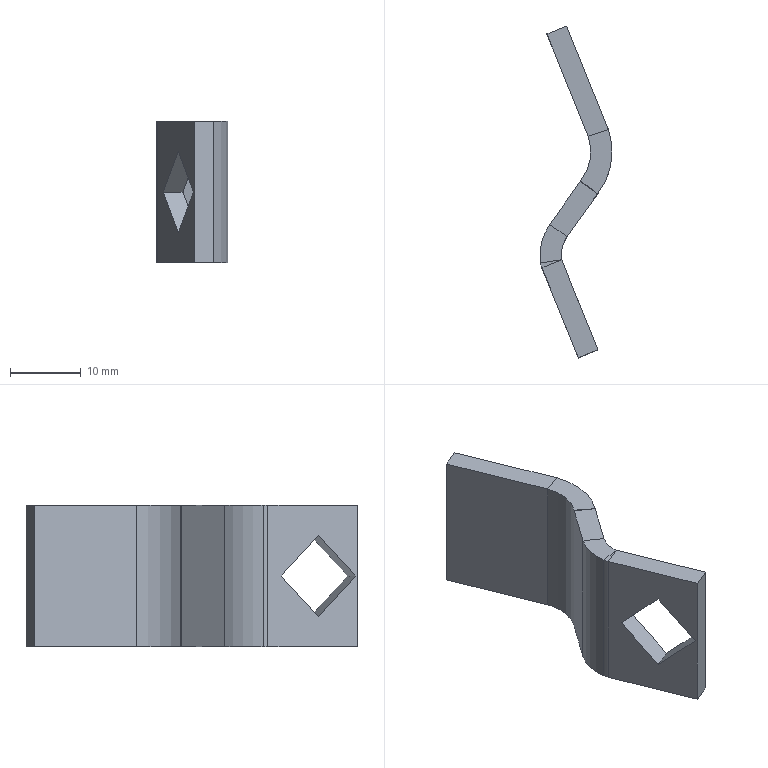Component | SolidWorks | RightDoorAssembly-1_LinkRodLock-1_Lock-1_Latch-1 | 1 solid | 38 faces | box 10.16 x 46.79 x 20 mm | volume 2800 mm3 | plane 28 | cylinder 10 | commonest cylinder face diameters 0.02 x3 6.02 x3 13.352 x1 14.968 x1 8.968 x1 19.352 x1
STEP:
#1=CARTESIAN_POINT('',(-12.644,16.473,37.449));
#2=VERTEX_POINT('',#1);
#3=CARTESIAN_POINT('',(-12.547,16.405,37.449));
#4=VERTEX_POINT('',#3);
#5=CARTESIAN_POINT('',(-12.644,16.473,37.449));
#6=DIRECTION('',(0.816,-0.578,0.));
#7=VECTOR('',#6,39.37);
#8=LINE('',#5,#7);
#9=EDGE_CURVE('',#2,#4,#8,.T.);
#10=ORIENTED_EDGE('',*,*,#9,.F.);
#11=CARTESIAN_POINT('',(-12.695,16.26,37.449));
#12=VERTEX_POINT('',#11);
#13=CARTESIAN_POINT('',(-12.403,16.303,37.449));
#14=DIRECTION('',(0.,0.,-1.));
#15=DIRECTION('',(0.3744,-0.9273,0.));
#16=AXIS2_PLACEMENT_3D('',#13,#14,#15);
#17=CIRCLE('',#16,0.2946);
#18=EDGE_CURVE('',#12,#2,#17,.T.);
#19=ORIENTED_EDGE('',*,*,#18,.F.);
#20=CARTESIAN_POINT('',(-12.578,16.277,37.449));
#21=VERTEX_POINT('',#20);
#22=CARTESIAN_POINT('',(-12.695,16.26,37.449));
#23=DIRECTION('',(0.9892,0.1467,0.));
#24=VECTOR('',#23,39.37);
#25=LINE('',#22,#24);
#26=EDGE_CURVE('',#12,#21,#25,.T.);
#27=ORIENTED_EDGE('',*,*,#26,.T.);
#28=CARTESIAN_POINT('',(-12.403,16.303,37.449));
#29=DIRECTION('',(0.,0.,-1.));
#30=DIRECTION('',(0.3744,-0.9273,0.));
#31=AXIS2_PLACEMENT_3D('',#28,#29,#30);
#32=CIRCLE('',#31,0.1765);
#33=EDGE_CURVE('',#21,#4,#32,.T.);
#34=ORIENTED_EDGE('',*,*,#33,.T.);
#35=EDGE_LOOP('',(#10,#19,#27,#34));
#36=FACE_OUTER_BOUND('',#35,.T.);
#37=CARTESIAN_POINT('',(-12.644,16.473,37.449));
#38=DIRECTION('',(-0.,-0.,1.));
#39=DIRECTION('',(0.3744,-0.9273,-0.));
#40=AXIS2_PLACEMENT_3D('',#37,#38,#39);
#41=PLANE('',#40);
#42=ADVANCED_FACE('',(#36),#41,.T.);
#43=CARTESIAN_POINT('',(-12.547,16.405,36.661));
#44=VERTEX_POINT('',#43);
#45=CARTESIAN_POINT('',(-12.644,16.473,36.661));
#46=VERTEX_POINT('',#45);
#47=CARTESIAN_POINT('',(-12.547,16.405,36.661));
#48=DIRECTION('',(-0.816,0.578,-0.));
#49=VECTOR('',#48,39.37);
#50=LINE('',#47,#49);
#51=EDGE_CURVE('',#44,#46,#50,.T.);
#52=ORIENTED_EDGE('',*,*,#51,.F.);
#53=CARTESIAN_POINT('',(-12.578,16.277,36.661));
#54=VERTEX_POINT('',#53);
#55=CARTESIAN_POINT('',(-12.403,16.303,36.661));
#56=DIRECTION('',(0.,0.,-1.));
#57=DIRECTION('',(0.3744,-0.9273,0.));
#58=AXIS2_PLACEMENT_3D('',#55,#56,#57);
#59=CIRCLE('',#58,0.1765);
#60=EDGE_CURVE('',#54,#44,#59,.T.);
#61=ORIENTED_EDGE('',*,*,#60,.F.);
#62=CARTESIAN_POINT('',(-12.695,16.26,36.661));
#63=VERTEX_POINT('',#62);
#64=CARTESIAN_POINT('',(-12.578,16.277,36.661));
#65=DIRECTION('',(-0.9892,-0.1467,-0.));
#66=VECTOR('',#65,39.37);
#67=LINE('',#64,#66);
#68=EDGE_CURVE('',#54,#63,#67,.T.);
#69=ORIENTED_EDGE('',*,*,#68,.T.);
#70=CARTESIAN_POINT('',(-12.403,16.303,36.661));
#71=DIRECTION('',(0.,0.,-1.));
#72=DIRECTION('',(0.3744,-0.9273,0.));
#73=AXIS2_PLACEMENT_3D('',#70,#71,#72);
#74=CIRCLE('',#73,0.2946);
#75=EDGE_CURVE('',#63,#46,#74,.T.);
#76=ORIENTED_EDGE('',*,*,#75,.T.);
#77=EDGE_LOOP('',(#52,#61,#69,#76));
#78=FACE_OUTER_BOUND('',#77,.T.);
#79=CARTESIAN_POINT('',(-12.547,16.405,36.661));
#80=DIRECTION('',(0.,0.,-1.));
#81=DIRECTION('',(-0.3744,0.9273,0.));
#82=AXIS2_PLACEMENT_3D('',#79,#80,#81);
#83=PLANE('',#82);
#84=ADVANCED_FACE('',(#78),#83,.T.);
#85=CARTESIAN_POINT('',(-12.43,16.963,37.449));
#86=VERTEX_POINT('',#85);
#87=CARTESIAN_POINT('',(-12.321,17.007,37.449));
#88=VERTEX_POINT('',#87);
#89=CARTESIAN_POINT('',(-12.43,16.963,37.449));
#90=DIRECTION('',(0.9273,0.3744,0.));
#91=VECTOR('',#90,39.37);
#92=LINE('',#89,#91);
#93=EDGE_CURVE('',#86,#88,#92,.T.);
#94=ORIENTED_EDGE('',*,*,#93,.F.);
#95=CARTESIAN_POINT('',(-12.43,16.963,37.449));
#96=VERTEX_POINT('',#95);
#97=CARTESIAN_POINT('',(-12.431,16.963,37.449));
#98=DIRECTION('',(-0.,-0.,1.));
#99=DIRECTION('',(0.3744,-0.9273,0.));
#100=AXIS2_PLACEMENT_3D('',#97,#98,#99);
#101=CIRCLE('',#100,0.0003937);
#102=EDGE_CURVE('',#96,#86,#101,.T.);
#103=ORIENTED_EDGE('',*,*,#102,.F.);
#104=CARTESIAN_POINT('',(-12.319,17.001,37.449));
#105=VERTEX_POINT('',#104);
#106=CARTESIAN_POINT('',(-12.319,17.001,37.449));
#107=DIRECTION('',(-0.9458,-0.3248,-0.));
#108=VECTOR('',#107,39.37);
#109=LINE('',#106,#108);
#110=EDGE_CURVE('',#105,#96,#109,.T.);
#111=ORIENTED_EDGE('',*,*,#110,.F.);
#112=CARTESIAN_POINT('',(-12.431,16.963,37.449));
#113=DIRECTION('',(-0.,-0.,1.));
#114=DIRECTION('',(0.3744,-0.9273,0.));
#115=AXIS2_PLACEMENT_3D('',#112,#113,#114);
#116=CIRCLE('',#115,0.1185);
#117=EDGE_CURVE('',#105,#88,#116,.T.);
#118=ORIENTED_EDGE('',*,*,#117,.T.);
#119=EDGE_LOOP('',(#94,#103,#111,#118));
#120=FACE_OUTER_BOUND('',#119,.T.);
#121=CARTESIAN_POINT('',(-12.43,16.963,37.449));
#122=DIRECTION('',(-0.,-0.,1.));
#123=DIRECTION('',(0.3744,-0.9273,-0.));
#124=AXIS2_PLACEMENT_3D('',#121,#122,#123);
#125=PLANE('',#124);
#126=ADVANCED_FACE('',(#120),#125,.T.);
#127=CARTESIAN_POINT('',(-12.66,17.531,37.449));
#128=VERTEX_POINT('',#127);
#129=CARTESIAN_POINT('',(-12.43,16.963,37.449));
#130=DIRECTION('',(-0.3744,0.9273,0.));
#131=VECTOR('',#130,39.37);
#132=LINE('',#129,#131);
#133=EDGE_CURVE('',#86,#128,#132,.T.);
#134=ORIENTED_EDGE('',*,*,#133,.F.);
#135=ORIENTED_EDGE('',*,*,#93,.T.);
#136=CARTESIAN_POINT('',(-12.55,17.575,37.449));
#137=VERTEX_POINT('',#136);
#138=CARTESIAN_POINT('',(-12.321,17.007,37.449));
#139=DIRECTION('',(-0.3744,0.9273,0.));
#140=VECTOR('',#139,39.37);
#141=LINE('',#138,#140);
#142=EDGE_CURVE('',#88,#137,#141,.T.);
#143=ORIENTED_EDGE('',*,*,#142,.T.);
#144=CARTESIAN_POINT('',(-12.66,17.531,37.449));
#145=DIRECTION('',(0.9273,0.3744,0.));
#146=VECTOR('',#145,39.37);
#147=LINE('',#144,#146);
#148=EDGE_CURVE('',#128,#137,#147,.T.);
#149=ORIENTED_EDGE('',*,*,#148,.F.);
#150=EDGE_LOOP('',(#134,#135,#143,#149));
#151=FACE_OUTER_BOUND('',#150,.T.);
#152=CARTESIAN_POINT('',(-12.319,17.001,37.449));
#153=DIRECTION('',(-0.,-0.,1.));
#154=DIRECTION('',(0.3744,-0.9273,-0.));
#155=AXIS2_PLACEMENT_3D('',#152,#153,#154);
#156=PLANE('',#155);
#157=ADVANCED_FACE('',(#151),#156,.T.);
#158=CARTESIAN_POINT('',(-12.43,16.963,36.661));
#159=VERTEX_POINT('',#158);
#160=CARTESIAN_POINT('',(-12.319,17.001,36.661));
#161=VERTEX_POINT('',#160);
#162=CARTESIAN_POINT('',(-12.43,16.963,36.661));
#163=DIRECTION('',(0.9458,0.3248,0.));
#164=VECTOR('',#163,39.37);
#165=LINE('',#162,#164);
#166=EDGE_CURVE('',#159,#161,#165,.T.);
#167=ORIENTED_EDGE('',*,*,#166,.F.);
#168=CARTESIAN_POINT('',(-12.43,16.963,36.661));
#169=VERTEX_POINT('',#168);
#170=CARTESIAN_POINT('',(-12.431,16.963,36.661));
#171=DIRECTION('',(-0.,-0.,1.));
#172=DIRECTION('',(0.3744,-0.9273,0.));
#173=AXIS2_PLACEMENT_3D('',#170,#171,#172);
#174=CIRCLE('',#173,0.0003937);
#175=EDGE_CURVE('',#159,#169,#174,.T.);
#176=ORIENTED_EDGE('',*,*,#175,.T.);
#177=CARTESIAN_POINT('',(-12.321,17.007,36.661));
#178=VERTEX_POINT('',#177);
#179=CARTESIAN_POINT('',(-12.321,17.007,36.661));
#180=DIRECTION('',(-0.9273,-0.3744,-0.));
#181=VECTOR('',#180,39.37);
#182=LINE('',#179,#181);
#183=EDGE_CURVE('',#178,#169,#182,.T.);
#184=ORIENTED_EDGE('',*,*,#183,.F.);
#185=CARTESIAN_POINT('',(-12.431,16.963,36.661));
#186=DIRECTION('',(-0.,-0.,1.));
#187=DIRECTION('',(0.3744,-0.9273,0.));
#188=AXIS2_PLACEMENT_3D('',#185,#186,#187);
#189=CIRCLE('',#188,0.1185);
#190=EDGE_CURVE('',#161,#178,#189,.T.);
#191=ORIENTED_EDGE('',*,*,#190,.F.);
#192=EDGE_LOOP('',(#167,#176,#184,#191));
#193=FACE_OUTER_BOUND('',#192,.T.);
#194=CARTESIAN_POINT('',(-12.43,16.963,36.661));
#195=DIRECTION('',(0.,0.,-1.));
#196=DIRECTION('',(-0.3744,0.9273,0.));
#197=AXIS2_PLACEMENT_3D('',#194,#195,#196);
#198=PLANE('',#197);
#199=ADVANCED_FACE('',(#193),#198,.T.);
#200=CARTESIAN_POINT('',(-12.472,16.716,36.661));
#201=VERTEX_POINT('',#200);
#202=CARTESIAN_POINT('',(-12.679,16.878,36.661));
#203=DIRECTION('',(-0.,-0.,1.));
#204=DIRECTION('',(0.3744,-0.9273,0.));
#205=AXIS2_PLACEMENT_3D('',#202,#203,#204);
#206=CIRCLE('',#205,0.2628);
#207=EDGE_CURVE('',#201,#159,#206,.T.);
#208=ORIENTED_EDGE('',*,*,#207,.T.);
#209=ORIENTED_EDGE('',*,*,#166,.T.);
#210=CARTESIAN_POINT('',(-12.379,16.643,36.661));
#211=VERTEX_POINT('',#210);
#212=CARTESIAN_POINT('',(-12.679,16.878,36.661));
#213=DIRECTION('',(-0.,-0.,1.));
#214=DIRECTION('',(0.3744,-0.9273,0.));
#215=AXIS2_PLACEMENT_3D('',#212,#213,#214);
#216=CIRCLE('',#215,0.3809);
#217=EDGE_CURVE('',#211,#161,#216,.T.);
#218=ORIENTED_EDGE('',*,*,#217,.F.);
#219=CARTESIAN_POINT('',(-12.379,16.643,36.661));
#220=DIRECTION('',(-0.7878,0.6159,-0.));
#221=VECTOR('',#220,39.37);
#222=LINE('',#219,#221);
#223=EDGE_CURVE('',#211,#201,#222,.T.);
#224=ORIENTED_EDGE('',*,*,#223,.T.);
#225=EDGE_LOOP('',(#208,#209,#218,#224));
#226=FACE_OUTER_BOUND('',#225,.T.);
#227=CARTESIAN_POINT('',(-12.321,17.007,36.661));
#228=DIRECTION('',(0.,0.,-1.));
#229=DIRECTION('',(-0.3744,0.9273,0.));
#230=AXIS2_PLACEMENT_3D('',#227,#228,#229);
#231=PLANE('',#230);
#232=ADVANCED_FACE('',(#226),#231,.T.);
#233=CARTESIAN_POINT('',(-12.472,16.716,37.449));
#234=VERTEX_POINT('',#233);
#235=CARTESIAN_POINT('',(-12.379,16.643,37.449));
#236=VERTEX_POINT('',#235);
#237=CARTESIAN_POINT('',(-12.472,16.716,37.449));
#238=DIRECTION('',(0.7878,-0.6159,0.));
#239=VECTOR('',#238,39.37);
#240=LINE('',#237,#239);
#241=EDGE_CURVE('',#234,#236,#240,.T.);
#242=ORIENTED_EDGE('',*,*,#241,.F.);
#243=CARTESIAN_POINT('',(-12.475,16.711,37.449));
#244=VERTEX_POINT('',#243);
#245=CARTESIAN_POINT('',(-12.378,16.643,37.449));
#246=DIRECTION('',(0.,0.,-1.));
#247=DIRECTION('',(0.3744,-0.9273,0.));
#248=AXIS2_PLACEMENT_3D('',#245,#246,#247);
#249=CIRCLE('',#248,0.1185);
#250=EDGE_CURVE('',#244,#234,#249,.T.);
#251=ORIENTED_EDGE('',*,*,#250,.F.);
#252=CARTESIAN_POINT('',(-12.379,16.643,37.449));
#253=VERTEX_POINT('',#252);
#254=CARTESIAN_POINT('',(-12.379,16.643,37.449));
#255=DIRECTION('',(-0.816,0.578,-0.));
#256=VECTOR('',#255,39.37);
#257=LINE('',#254,#256);
#258=EDGE_CURVE('',#253,#244,#257,.T.);
#259=ORIENTED_EDGE('',*,*,#258,.F.);
#260=CARTESIAN_POINT('',(-12.378,16.643,37.449));
#261=DIRECTION('',(0.,0.,-1.));
#262=DIRECTION('',(0.3744,-0.9273,0.));
#263=AXIS2_PLACEMENT_3D('',#260,#261,#262);
#264=CIRCLE('',#263,0.0003937);
#265=EDGE_CURVE('',#253,#236,#264,.T.);
#266=ORIENTED_EDGE('',*,*,#265,.T.);
#267=EDGE_LOOP('',(#242,#251,#259,#266));
#268=FACE_OUTER_BOUND('',#267,.T.);
#269=CARTESIAN_POINT('',(-12.472,16.716,37.449));
#270=DIRECTION('',(-0.,-0.,1.));
#271=DIRECTION('',(0.3744,-0.9273,-0.));
#272=AXIS2_PLACEMENT_3D('',#269,#270,#271);
#273=PLANE('',#272);
#274=ADVANCED_FACE('',(#268),#273,.T.);
#275=CARTESIAN_POINT('',(-12.679,16.878,37.449));
#276=DIRECTION('',(-0.,-0.,1.));
#277=DIRECTION('',(0.3744,-0.9273,0.));
#278=AXIS2_PLACEMENT_3D('',#275,#276,#277);
#279=CIRCLE('',#278,0.2628);
#280=EDGE_CURVE('',#234,#96,#279,.T.);
#281=ORIENTED_EDGE('',*,*,#280,.F.);
#282=ORIENTED_EDGE('',*,*,#241,.T.);
#283=CARTESIAN_POINT('',(-12.679,16.878,37.449));
#284=DIRECTION('',(-0.,-0.,1.));
#285=DIRECTION('',(0.3744,-0.9273,0.));
#286=AXIS2_PLACEMENT_3D('',#283,#284,#285);
#287=CIRCLE('',#286,0.3809);
#288=EDGE_CURVE('',#236,#105,#287,.T.);
#289=ORIENTED_EDGE('',*,*,#288,.T.);
#290=ORIENTED_EDGE('',*,*,#110,.T.);
#291=EDGE_LOOP('',(#281,#282,#289,#290));
#292=FACE_OUTER_BOUND('',#291,.T.);
#293=CARTESIAN_POINT('',(-12.379,16.643,37.449));
#294=DIRECTION('',(-0.,-0.,1.));
#295=DIRECTION('',(0.3744,-0.9273,-0.));
#296=AXIS2_PLACEMENT_3D('',#293,#294,#295);
#297=PLANE('',#296);
#298=ADVANCED_FACE('',(#292),#297,.T.);
#299=CARTESIAN_POINT('',(-12.475,16.711,36.661));
#300=VERTEX_POINT('',#299);
#301=CARTESIAN_POINT('',(-12.379,16.643,36.661));
#302=VERTEX_POINT('',#301);
#303=CARTESIAN_POINT('',(-12.475,16.711,36.661));
#304=DIRECTION('',(0.816,-0.578,0.));
#305=VECTOR('',#304,39.37);
#306=LINE('',#303,#305);
#307=EDGE_CURVE('',#300,#302,#306,.T.);
#308=ORIENTED_EDGE('',*,*,#307,.F.);
#309=CARTESIAN_POINT('',(-12.378,16.643,36.661));
#310=DIRECTION('',(0.,0.,-1.));
#311=DIRECTION('',(0.3744,-0.9273,0.));
#312=AXIS2_PLACEMENT_3D('',#309,#310,#311);
#313=CIRCLE('',#312,0.1185);
#314=EDGE_CURVE('',#300,#201,#313,.T.);
#315=ORIENTED_EDGE('',*,*,#314,.T.);
#316=ORIENTED_EDGE('',*,*,#223,.F.);
#317=CARTESIAN_POINT('',(-12.378,16.643,36.661));
#318=DIRECTION('',(0.,0.,-1.));
#319=DIRECTION('',(0.3744,-0.9273,0.));
#320=AXIS2_PLACEMENT_3D('',#317,#318,#319);
#321=CIRCLE('',#320,0.0003937);
#322=EDGE_CURVE('',#302,#211,#321,.T.);
#323=ORIENTED_EDGE('',*,*,#322,.F.);
#324=EDGE_LOOP('',(#308,#315,#316,#323));
#325=FACE_OUTER_BOUND('',#324,.T.);
#326=CARTESIAN_POINT('',(-12.475,16.711,36.661));
#327=DIRECTION('',(0.,0.,-1.));
#328=DIRECTION('',(-0.3744,0.9273,0.));
#329=AXIS2_PLACEMENT_3D('',#326,#327,#328);
#330=PLANE('',#329);
#331=ADVANCED_FACE('',(#325),#330,.T.);
#332=CARTESIAN_POINT('',(-12.473,16.714,36.661));
#333=DIRECTION('',(0.578,0.816,0.));
#334=VECTOR('',#333,39.37);
#335=LINE('',#332,#334);
#336=EDGE_CURVE('',#46,#300,#335,.T.);
#337=ORIENTED_EDGE('',*,*,#336,.T.);
#338=ORIENTED_EDGE('',*,*,#307,.T.);
#339=CARTESIAN_POINT('',(-12.377,16.645,36.661));
#340=DIRECTION('',(0.578,0.816,0.));
#341=VECTOR('',#340,39.37);
#342=LINE('',#339,#341);
#343=EDGE_CURVE('',#44,#302,#342,.T.);
#344=ORIENTED_EDGE('',*,*,#343,.F.);
#345=ORIENTED_EDGE('',*,*,#51,.T.);
#346=EDGE_LOOP('',(#337,#338,#344,#345));
#347=FACE_OUTER_BOUND('',#346,.T.);
#348=CARTESIAN_POINT('',(-12.379,16.643,36.661));
#349=DIRECTION('',(0.,0.,-1.));
#350=DIRECTION('',(-0.3744,0.9273,0.));
#351=AXIS2_PLACEMENT_3D('',#348,#349,#350);
#352=PLANE('',#351);
#353=ADVANCED_FACE('',(#347),#352,.T.);
#354=ORIENTED_EDGE('',*,*,#26,.F.);
#355=CARTESIAN_POINT('',(-12.687,16.233,37.449));
#356=VERTEX_POINT('',#355);
#357=CARTESIAN_POINT('',(-12.577,16.277,37.449));
#358=DIRECTION('',(0.,0.,-1.));
#359=DIRECTION('',(-0.3744,0.9273,0.));
#360=AXIS2_PLACEMENT_3D('',#357,#358,#359);
#361=CIRCLE('',#360,0.1185);
#362=EDGE_CURVE('',#356,#12,#361,.T.);
#363=ORIENTED_EDGE('',*,*,#362,.F.);
#364=CARTESIAN_POINT('',(-12.578,16.277,37.449));
#365=VERTEX_POINT('',#364);
#366=CARTESIAN_POINT('',(-12.578,16.277,37.449));
#367=DIRECTION('',(-0.9273,-0.3744,-0.));
#368=VECTOR('',#367,39.37);
#369=LINE('',#366,#368);
#370=EDGE_CURVE('',#365,#356,#369,.T.);
#371=ORIENTED_EDGE('',*,*,#370,.F.);
#372=CARTESIAN_POINT('',(-12.577,16.277,37.449));
#373=DIRECTION('',(0.,0.,-1.));
#374=DIRECTION('',(0.3744,-0.9273,0.));
#375=AXIS2_PLACEMENT_3D('',#372,#373,#374);
#376=CIRCLE('',#375,0.0003937);
#377=EDGE_CURVE('',#365,#21,#376,.T.);
#378=ORIENTED_EDGE('',*,*,#377,.T.);
#379=EDGE_LOOP('',(#354,#363,#371,#378));
#380=FACE_OUTER_BOUND('',#379,.T.);
#381=CARTESIAN_POINT('',(-12.695,16.26,37.449));
#382=DIRECTION('',(-0.,-0.,1.));
#383=DIRECTION('',(0.3744,-0.9273,-0.));
#384=AXIS2_PLACEMENT_3D('',#381,#382,#383);
#385=PLANE('',#384);
#386=ADVANCED_FACE('',(#380),#385,.T.);
#387=CARTESIAN_POINT('',(-12.473,16.714,37.449));
#388=DIRECTION('',(0.578,0.816,0.));
#389=VECTOR('',#388,39.37);
#390=LINE('',#387,#389);
#391=EDGE_CURVE('',#2,#244,#390,.T.);
#392=ORIENTED_EDGE('',*,*,#391,.F.);
#393=ORIENTED_EDGE('',*,*,#9,.T.);
#394=CARTESIAN_POINT('',(-12.377,16.645,37.449));
#395=DIRECTION('',(0.578,0.816,0.));
#396=VECTOR('',#395,39.37);
#397=LINE('',#394,#396);
#398=EDGE_CURVE('',#4,#253,#397,.T.);
#399=ORIENTED_EDGE('',*,*,#398,.T.);
#400=ORIENTED_EDGE('',*,*,#258,.T.);
#401=EDGE_LOOP('',(#392,#393,#399,#400));
#402=FACE_OUTER_BOUND('',#401,.T.);
#403=CARTESIAN_POINT('',(-12.578,16.277,37.449));
#404=DIRECTION('',(-0.,-0.,1.));
#405=DIRECTION('',(0.3744,-0.9273,-0.));
#406=AXIS2_PLACEMENT_3D('',#403,#404,#405);
#407=PLANE('',#406);
#408=ADVANCED_FACE('',(#402),#407,.T.);
#409=CARTESIAN_POINT('',(-12.687,16.233,36.661));
#410=VERTEX_POINT('',#409);
#411=CARTESIAN_POINT('',(-12.578,16.277,36.661));
#412=VERTEX_POINT('',#411);
#413=CARTESIAN_POINT('',(-12.687,16.233,36.661));
#414=DIRECTION('',(0.9273,0.3744,0.));
#415=VECTOR('',#414,39.37);
#416=LINE('',#413,#415);
#417=EDGE_CURVE('',#410,#412,#416,.T.);
#418=ORIENTED_EDGE('',*,*,#417,.F.);
#419=CARTESIAN_POINT('',(-12.577,16.277,36.661));
#420=DIRECTION('',(0.,0.,-1.));
#421=DIRECTION('',(-0.3744,0.9273,0.));
#422=AXIS2_PLACEMENT_3D('',#419,#420,#421);
#423=CIRCLE('',#422,0.1185);
#424=EDGE_CURVE('',#410,#63,#423,.T.);
#425=ORIENTED_EDGE('',*,*,#424,.T.);
#426=ORIENTED_EDGE('',*,*,#68,.F.);
#427=CARTESIAN_POINT('',(-12.577,16.277,36.661));
#428=DIRECTION('',(0.,0.,-1.));
#429=DIRECTION('',(0.3744,-0.9273,0.));
#430=AXIS2_PLACEMENT_3D('',#427,#428,#429);
#431=CIRCLE('',#430,0.0003937);
#432=EDGE_CURVE('',#412,#54,#431,.T.);
#433=ORIENTED_EDGE('',*,*,#432,.F.);
#434=EDGE_LOOP('',(#418,#425,#426,#433));
#435=FACE_OUTER_BOUND('',#434,.T.);
#436=CARTESIAN_POINT('',(-12.687,16.233,36.661));
#437=DIRECTION('',(0.,0.,-1.));
#438=DIRECTION('',(-0.3744,0.9273,0.));
#439=AXIS2_PLACEMENT_3D('',#436,#437,#438);
#440=PLANE('',#439);
#441=ADVANCED_FACE('',(#435),#440,.T.);
#442=CARTESIAN_POINT('',(-12.486,15.733,36.661));
#443=VERTEX_POINT('',#442);
#444=CARTESIAN_POINT('',(-12.486,15.733,36.661));
#445=DIRECTION('',(-0.3744,0.9273,0.));
#446=VECTOR('',#445,39.37);
#447=LINE('',#444,#446);
#448=EDGE_CURVE('',#443,#410,#447,.T.);
#449=ORIENTED_EDGE('',*,*,#448,.T.);
#450=ORIENTED_EDGE('',*,*,#417,.T.);
#451=CARTESIAN_POINT('',(-12.376,15.777,36.661));
#452=VERTEX_POINT('',#451);
#453=CARTESIAN_POINT('',(-12.376,15.777,36.661));
#454=DIRECTION('',(-0.3744,0.9273,0.));
#455=VECTOR('',#454,39.37);
#456=LINE('',#453,#455);
#457=EDGE_CURVE('',#452,#412,#456,.T.);
#458=ORIENTED_EDGE('',*,*,#457,.F.);
#459=CARTESIAN_POINT('',(-12.376,15.777,36.661));
#460=DIRECTION('',(-0.9273,-0.3744,-0.));
#461=VECTOR('',#460,39.37);
#462=LINE('',#459,#461);
#463=EDGE_CURVE('',#452,#443,#462,.T.);
#464=ORIENTED_EDGE('',*,*,#463,.T.);
#465=EDGE_LOOP('',(#449,#450,#458,#464));
#466=FACE_OUTER_BOUND('',#465,.T.);
#467=CARTESIAN_POINT('',(-12.578,16.277,36.661));
#468=DIRECTION('',(0.,0.,-1.));
#469=DIRECTION('',(-0.3744,0.9273,0.));
#470=AXIS2_PLACEMENT_3D('',#467,#468,#469);
#471=PLANE('',#470);
#472=ADVANCED_FACE('',(#466),#471,.T.);
#473=CARTESIAN_POINT('',(-12.55,17.575,36.661));
#474=VERTEX_POINT('',#473);
#475=CARTESIAN_POINT('',(-12.321,17.007,36.661));
#476=DIRECTION('',(-0.3744,0.9273,0.));
#477=VECTOR('',#476,39.37);
#478=LINE('',#475,#477);
#479=EDGE_CURVE('',#178,#474,#478,.T.);
#480=ORIENTED_EDGE('',*,*,#479,.T.);
#481=CARTESIAN_POINT('',(-12.55,17.575,37.449));
#482=DIRECTION('',(0.,0.,-1.));
#483=VECTOR('',#482,39.37);
#484=LINE('',#481,#483);
#485=EDGE_CURVE('',#137,#474,#484,.T.);
#486=ORIENTED_EDGE('',*,*,#485,.F.);
#487=ORIENTED_EDGE('',*,*,#142,.F.);
#488=CARTESIAN_POINT('',(-12.321,17.007,37.449));
#489=DIRECTION('',(0.,0.,-1.));
#490=VECTOR('',#489,39.37);
#491=LINE('',#488,#490);
#492=EDGE_CURVE('',#88,#178,#491,.T.);
#493=ORIENTED_EDGE('',*,*,#492,.T.);
#494=EDGE_LOOP('',(#480,#486,#487,#493));
#495=FACE_OUTER_BOUND('',#494,.T.);
#496=CARTESIAN_POINT('',(-12.321,17.007,37.449));
#497=DIRECTION('',(-0.9273,-0.3744,-0.));
#498=DIRECTION('',(0.3744,-0.9273,-0.));
#499=AXIS2_PLACEMENT_3D('',#496,#497,#498);
#500=PLANE('',#499);
#501=ADVANCED_FACE('',(#495),#500,.F.);
#502=CARTESIAN_POINT('',(-12.66,17.531,36.661));
#503=VERTEX_POINT('',#502);
#504=CARTESIAN_POINT('',(-12.66,17.531,36.661));
#505=DIRECTION('',(0.9273,0.3744,0.));
#506=VECTOR('',#505,39.37);
#507=LINE('',#504,#506);
#508=EDGE_CURVE('',#503,#474,#507,.T.);
#509=ORIENTED_EDGE('',*,*,#508,.F.);
#510=CARTESIAN_POINT('',(-12.66,17.531,37.449));
#511=DIRECTION('',(0.,0.,-1.));
#512=VECTOR('',#511,39.37);
#513=LINE('',#510,#512);
#514=EDGE_CURVE('',#128,#503,#513,.T.);
#515=ORIENTED_EDGE('',*,*,#514,.F.);
#516=ORIENTED_EDGE('',*,*,#148,.T.);
#517=ORIENTED_EDGE('',*,*,#485,.T.);
#518=EDGE_LOOP('',(#509,#515,#516,#517));
#519=FACE_OUTER_BOUND('',#518,.T.);
#520=CARTESIAN_POINT('',(-12.66,17.531,37.449));
#521=DIRECTION('',(-0.3744,0.9273,0.));
#522=DIRECTION('',(-0.9273,-0.3744,-0.));
#523=AXIS2_PLACEMENT_3D('',#520,#521,#522);
#524=PLANE('',#523);
#525=ADVANCED_FACE('',(#519),#524,.T.);
#526=CARTESIAN_POINT('',(-12.43,16.963,36.661));
#527=DIRECTION('',(-0.3744,0.9273,0.));
#528=VECTOR('',#527,39.37);
#529=LINE('',#526,#528);
#530=EDGE_CURVE('',#169,#503,#529,.T.);
#531=ORIENTED_EDGE('',*,*,#530,.F.);
#532=CARTESIAN_POINT('',(-12.43,16.963,37.449));
#533=DIRECTION('',(0.,0.,-1.));
#534=VECTOR('',#533,39.37);
#535=LINE('',#532,#534);
#536=EDGE_CURVE('',#86,#169,#535,.T.);
#537=ORIENTED_EDGE('',*,*,#536,.F.);
#538=ORIENTED_EDGE('',*,*,#133,.T.);
#539=ORIENTED_EDGE('',*,*,#514,.T.);
#540=EDGE_LOOP('',(#531,#537,#538,#539));
#541=FACE_OUTER_BOUND('',#540,.T.);
#542=CARTESIAN_POINT('',(-12.43,16.963,37.449));
#543=DIRECTION('',(-0.9273,-0.3744,-0.));
#544=DIRECTION('',(0.3744,-0.9273,-0.));
#545=AXIS2_PLACEMENT_3D('',#542,#543,#544);
#546=PLANE('',#545);
#547=ADVANCED_FACE('',(#541),#546,.T.);
#548=ORIENTED_EDGE('',*,*,#175,.F.);
#549=CARTESIAN_POINT('',(-12.43,16.963,37.449));
#550=DIRECTION('',(0.,0.,-1.));
#551=VECTOR('',#550,39.37);
#552=LINE('',#549,#551);
#553=EDGE_CURVE('',#96,#159,#552,.T.);
#554=ORIENTED_EDGE('',*,*,#553,.F.);
#555=ORIENTED_EDGE('',*,*,#102,.T.);
#556=ORIENTED_EDGE('',*,*,#536,.T.);
#557=EDGE_LOOP('',(#548,#554,#555,#556));
#558=FACE_OUTER_BOUND('',#557,.T.);
#559=CARTESIAN_POINT('',(-12.431,16.963,37.449));
#560=DIRECTION('',(0.,0.,-1.));
#561=DIRECTION('',(-0.3744,0.9273,0.));
#562=AXIS2_PLACEMENT_3D('',#559,#560,#561);
#563=CYLINDRICAL_SURFACE('',#562,0.0003937);
#564=ADVANCED_FACE('',(#558),#563,.F.);
#565=ORIENTED_EDGE('',*,*,#207,.F.);
#566=CARTESIAN_POINT('',(-12.472,16.716,37.449));
#567=DIRECTION('',(0.,0.,-1.));
#568=VECTOR('',#567,39.37);
#569=LINE('',#566,#568);
#570=EDGE_CURVE('',#234,#201,#569,.T.);
#571=ORIENTED_EDGE('',*,*,#570,.F.);
#572=ORIENTED_EDGE('',*,*,#280,.T.);
#573=ORIENTED_EDGE('',*,*,#553,.T.);
#574=EDGE_LOOP('',(#565,#571,#572,#573));
#575=FACE_OUTER_BOUND('',#574,.T.);
#576=CARTESIAN_POINT('',(-12.679,16.878,37.449));
#577=DIRECTION('',(0.,0.,-1.));
#578=DIRECTION('',(-0.3744,0.9273,0.));
#579=AXIS2_PLACEMENT_3D('',#576,#577,#578);
#580=CYLINDRICAL_SURFACE('',#579,0.2628);
#581=ADVANCED_FACE('',(#575),#580,.F.);
#582=ORIENTED_EDGE('',*,*,#314,.F.);
#583=CARTESIAN_POINT('',(-12.475,16.711,37.449));
#584=DIRECTION('',(0.,0.,-1.));
#585=VECTOR('',#584,39.37);
#586=LINE('',#583,#585);
#587=EDGE_CURVE('',#244,#300,#586,.T.);
#588=ORIENTED_EDGE('',*,*,#587,.F.);
#589=ORIENTED_EDGE('',*,*,#250,.T.);
#590=ORIENTED_EDGE('',*,*,#570,.T.);
#591=EDGE_LOOP('',(#582,#588,#589,#590));
#592=FACE_OUTER_BOUND('',#591,.T.);
#593=CARTESIAN_POINT('',(-12.378,16.643,37.449));
#594=DIRECTION('',(0.,0.,-1.));
#595=DIRECTION('',(-0.3744,0.9273,0.));
#596=AXIS2_PLACEMENT_3D('',#593,#594,#595);
#597=CYLINDRICAL_SURFACE('',#596,0.1185);
#598=ADVANCED_FACE('',(#592),#597,.T.);
#599=ORIENTED_EDGE('',*,*,#336,.F.);
#600=CARTESIAN_POINT('',(-12.644,16.473,37.449));
#601=DIRECTION('',(0.,0.,-1.));
#602=VECTOR('',#601,39.37);
#603=LINE('',#600,#602);
#604=EDGE_CURVE('',#2,#46,#603,.T.);
#605=ORIENTED_EDGE('',*,*,#604,.F.);
#606=ORIENTED_EDGE('',*,*,#391,.T.);
#607=ORIENTED_EDGE('',*,*,#587,.T.);
#608=EDGE_LOOP('',(#599,#605,#606,#607));
#609=FACE_OUTER_BOUND('',#608,.T.);
#610=CARTESIAN_POINT('',(-12.473,16.714,37.449));
#611=DIRECTION('',(-0.816,0.578,-0.));
#612=DIRECTION('',(-0.578,-0.816,-0.));
#613=AXIS2_PLACEMENT_3D('',#610,#611,#612);
#614=PLANE('',#613);
#615=ADVANCED_FACE('',(#609),#614,.T.);
#616=ORIENTED_EDGE('',*,*,#75,.F.);
#617=CARTESIAN_POINT('',(-12.695,16.26,37.449));
#618=DIRECTION('',(0.,0.,-1.));
#619=VECTOR('',#618,39.37);
#620=LINE('',#617,#619);
#621=EDGE_CURVE('',#12,#63,#620,.T.);
#622=ORIENTED_EDGE('',*,*,#621,.F.);
#623=ORIENTED_EDGE('',*,*,#18,.T.);
#624=ORIENTED_EDGE('',*,*,#604,.T.);
#625=EDGE_LOOP('',(#616,#622,#623,#624));
#626=FACE_OUTER_BOUND('',#625,.T.);
#627=CARTESIAN_POINT('',(-12.403,16.303,37.449));
#628=DIRECTION('',(0.,0.,-1.));
#629=DIRECTION('',(-0.3744,0.9273,0.));
#630=AXIS2_PLACEMENT_3D('',#627,#628,#629);
#631=CYLINDRICAL_SURFACE('',#630,0.2946);
#632=ADVANCED_FACE('',(#626),#631,.T.);
#633=ORIENTED_EDGE('',*,*,#424,.F.);
#634=CARTESIAN_POINT('',(-12.687,16.233,37.449));
#635=DIRECTION('',(0.,0.,-1.));
#636=VECTOR('',#635,39.37);
#637=LINE('',#634,#636);
#638=EDGE_CURVE('',#356,#410,#637,.T.);
#639=ORIENTED_EDGE('',*,*,#638,.F.);
#640=ORIENTED_EDGE('',*,*,#362,.T.);
#641=ORIENTED_EDGE('',*,*,#621,.T.);
#642=EDGE_LOOP('',(#633,#639,#640,#641));
#643=FACE_OUTER_BOUND('',#642,.T.);
#644=CARTESIAN_POINT('',(-12.577,16.277,37.449));
#645=DIRECTION('',(0.,0.,-1.));
#646=DIRECTION('',(-0.3744,0.9273,0.));
#647=AXIS2_PLACEMENT_3D('',#644,#645,#646);
#648=CYLINDRICAL_SURFACE('',#647,0.1185);
#649=ADVANCED_FACE('',(#643),#648,.T.);
#650=CARTESIAN_POINT('',(-12.657,16.159,37.055));
#651=VERTEX_POINT('',#650);
#652=CARTESIAN_POINT('',(-12.574,15.952,36.832));
#653=VERTEX_POINT('',#652);
#654=CARTESIAN_POINT('',(-12.645,16.128,37.023));
#655=DIRECTION('',(0.2647,-0.6557,-0.7071));
#656=VECTOR('',#655,39.37);
#657=LINE('',#654,#656);
#658=EDGE_CURVE('',#651,#653,#657,.T.);
#659=ORIENTED_EDGE('',*,*,#658,.F.);
#660=CARTESIAN_POINT('',(-12.574,15.952,37.278));
#661=VERTEX_POINT('',#660);
#662=CARTESIAN_POINT('',(-12.498,15.763,37.481));
#663=DIRECTION('',(-0.2647,0.6557,-0.7071));
#664=VECTOR('',#663,39.37);
#665=LINE('',#662,#664);
#666=EDGE_CURVE('',#661,#651,#665,.T.);
#667=ORIENTED_EDGE('',*,*,#666,.F.);
#668=CARTESIAN_POINT('',(-12.491,15.746,37.055));
#669=VERTEX_POINT('',#668);
#670=CARTESIAN_POINT('',(-12.562,15.922,37.245));
#671=DIRECTION('',(-0.2647,0.6557,0.7071));
#672=VECTOR('',#671,39.37);
#673=LINE('',#670,#672);
#674=EDGE_CURVE('',#669,#661,#673,.T.);
#675=ORIENTED_EDGE('',*,*,#674,.F.);
#676=CARTESIAN_POINT('',(-12.414,15.557,37.259));
#677=DIRECTION('',(0.2647,-0.6557,0.7071));
#678=VECTOR('',#677,39.37);
#679=LINE('',#676,#678);
#680=EDGE_CURVE('',#653,#669,#679,.T.);
#681=ORIENTED_EDGE('',*,*,#680,.F.);
#682=EDGE_LOOP('',(#659,#667,#675,#681));
#683=FACE_BOUND('',#682,.T.);
#684=ORIENTED_EDGE('',*,*,#448,.F.);
#685=CARTESIAN_POINT('',(-12.486,15.733,37.449));
#686=VERTEX_POINT('',#685);
#687=CARTESIAN_POINT('',(-12.486,15.733,37.449));
#688=DIRECTION('',(0.,0.,-1.));
#689=VECTOR('',#688,39.37);
#690=LINE('',#687,#689);
#691=EDGE_CURVE('',#686,#443,#690,.T.);
#692=ORIENTED_EDGE('',*,*,#691,.F.);
#693=CARTESIAN_POINT('',(-12.486,15.733,37.449));
#694=DIRECTION('',(-0.3744,0.9273,0.));
#695=VECTOR('',#694,39.37);
#696=LINE('',#693,#695);
#697=EDGE_CURVE('',#686,#356,#696,.T.);
#698=ORIENTED_EDGE('',*,*,#697,.T.);
#699=ORIENTED_EDGE('',*,*,#638,.T.);
#700=EDGE_LOOP('',(#684,#692,#698,#699));
#701=FACE_OUTER_BOUND('',#700,.T.);
#702=CARTESIAN_POINT('',(-12.486,15.733,37.449));
#703=DIRECTION('',(-0.9273,-0.3744,-0.));
#704=DIRECTION('',(0.3744,-0.9273,-0.));
#705=AXIS2_PLACEMENT_3D('',#702,#703,#704);
#706=PLANE('',#705);
#707=ADVANCED_FACE('',(#683,#701),#706,.T.);
#708=ORIENTED_EDGE('',*,*,#463,.F.);
#709=CARTESIAN_POINT('',(-12.376,15.777,37.449));
#710=VERTEX_POINT('',#709);
#711=CARTESIAN_POINT('',(-12.376,15.777,37.449));
#712=DIRECTION('',(0.,0.,-1.));
#713=VECTOR('',#712,39.37);
#714=LINE('',#711,#713);
#715=EDGE_CURVE('',#710,#452,#714,.T.);
#716=ORIENTED_EDGE('',*,*,#715,.F.);
#717=CARTESIAN_POINT('',(-12.376,15.777,37.449));
#718=DIRECTION('',(-0.9273,-0.3744,-0.));
#719=VECTOR('',#718,39.37);
#720=LINE('',#717,#719);
#721=EDGE_CURVE('',#710,#686,#720,.T.);
#722=ORIENTED_EDGE('',*,*,#721,.T.);
#723=ORIENTED_EDGE('',*,*,#691,.T.);
#724=EDGE_LOOP('',(#708,#716,#722,#723));
#725=FACE_OUTER_BOUND('',#724,.T.);
#726=CARTESIAN_POINT('',(-12.376,15.777,37.449));
#727=DIRECTION('',(0.3744,-0.9273,-0.));
#728=DIRECTION('',(0.9273,0.3744,0.));
#729=AXIS2_PLACEMENT_3D('',#726,#727,#728);
#730=PLANE('',#729);
#731=ADVANCED_FACE('',(#725),#730,.T.);
#732=CARTESIAN_POINT('',(-12.548,16.203,37.055));
#733=VERTEX_POINT('',#732);
#734=CARTESIAN_POINT('',(-12.465,15.996,37.278));
#735=VERTEX_POINT('',#734);
#736=CARTESIAN_POINT('',(-12.548,16.203,37.055));
#737=DIRECTION('',(0.2647,-0.6557,0.7071));
#738=VECTOR('',#737,39.37);
#739=LINE('',#736,#738);
#740=EDGE_CURVE('',#733,#735,#739,.T.);
#741=ORIENTED_EDGE('',*,*,#740,.F.);
#742=CARTESIAN_POINT('',(-12.465,15.996,36.832));
#743=VERTEX_POINT('',#742);
#744=CARTESIAN_POINT('',(-12.465,15.996,36.832));
#745=DIRECTION('',(-0.2647,0.6557,0.7071));
#746=VECTOR('',#745,39.37);
#747=LINE('',#744,#746);
#748=EDGE_CURVE('',#743,#733,#747,.T.);
#749=ORIENTED_EDGE('',*,*,#748,.F.);
#750=CARTESIAN_POINT('',(-12.381,15.79,37.055));
#751=VERTEX_POINT('',#750);
#752=CARTESIAN_POINT('',(-12.465,15.996,36.832));
#753=DIRECTION('',(-0.2647,0.6557,-0.7071));
#754=VECTOR('',#753,39.37);
#755=LINE('',#752,#754);
#756=EDGE_CURVE('',#751,#743,#755,.T.);
#757=ORIENTED_EDGE('',*,*,#756,.F.);
#758=CARTESIAN_POINT('',(-12.381,15.79,37.055));
#759=DIRECTION('',(0.2647,-0.6557,-0.7071));
#760=VECTOR('',#759,39.37);
#761=LINE('',#758,#760);
#762=EDGE_CURVE('',#735,#751,#761,.T.);
#763=ORIENTED_EDGE('',*,*,#762,.F.);
#764=EDGE_LOOP('',(#741,#749,#757,#763));
#765=FACE_BOUND('',#764,.T.);
#766=ORIENTED_EDGE('',*,*,#457,.T.);
#767=CARTESIAN_POINT('',(-12.578,16.277,37.449));
#768=DIRECTION('',(0.,0.,-1.));
#769=VECTOR('',#768,39.37);
#770=LINE('',#767,#769);
#771=EDGE_CURVE('',#365,#412,#770,.T.);
#772=ORIENTED_EDGE('',*,*,#771,.F.);
#773=CARTESIAN_POINT('',(-12.376,15.777,37.449));
#774=DIRECTION('',(-0.3744,0.9273,0.));
#775=VECTOR('',#774,39.37);
#776=LINE('',#773,#775);
#777=EDGE_CURVE('',#710,#365,#776,.T.);
#778=ORIENTED_EDGE('',*,*,#777,.F.);
#779=ORIENTED_EDGE('',*,*,#715,.T.);
#780=EDGE_LOOP('',(#766,#772,#778,#779));
#781=FACE_OUTER_BOUND('',#780,.T.);
#782=CARTESIAN_POINT('',(-12.376,15.777,37.449));
#783=DIRECTION('',(-0.9273,-0.3744,-0.));
#784=DIRECTION('',(0.3744,-0.9273,-0.));
#785=AXIS2_PLACEMENT_3D('',#782,#783,#784);
#786=PLANE('',#785);
#787=ADVANCED_FACE('',(#765,#781),#786,.F.);
#788=ORIENTED_EDGE('',*,*,#432,.T.);
#789=CARTESIAN_POINT('',(-12.578,16.277,37.449));
#790=DIRECTION('',(0.,0.,-1.));
#791=VECTOR('',#790,39.37);
#792=LINE('',#789,#791);
#793=EDGE_CURVE('',#21,#54,#792,.T.);
#794=ORIENTED_EDGE('',*,*,#793,.F.);
#795=ORIENTED_EDGE('',*,*,#377,.F.);
#796=ORIENTED_EDGE('',*,*,#771,.T.);
#797=EDGE_LOOP('',(#788,#794,#795,#796));
#798=FACE_OUTER_BOUND('',#797,.T.);
#799=CARTESIAN_POINT('',(-12.577,16.277,37.449));
#800=DIRECTION('',(0.,0.,-1.));
#801=DIRECTION('',(-0.3744,0.9273,0.));
#802=AXIS2_PLACEMENT_3D('',#799,#800,#801);
#803=CYLINDRICAL_SURFACE('',#802,0.0003937);
#804=ADVANCED_FACE('',(#798),#803,.F.);
#805=ORIENTED_EDGE('',*,*,#60,.T.);
#806=CARTESIAN_POINT('',(-12.547,16.405,37.449));
#807=DIRECTION('',(0.,0.,-1.));
#808=VECTOR('',#807,39.37);
#809=LINE('',#806,#808);
#810=EDGE_CURVE('',#4,#44,#809,.T.);
#811=ORIENTED_EDGE('',*,*,#810,.F.);
#812=ORIENTED_EDGE('',*,*,#33,.F.);
#813=ORIENTED_EDGE('',*,*,#793,.T.);
#814=EDGE_LOOP('',(#805,#811,#812,#813));
#815=FACE_OUTER_BOUND('',#814,.T.);
#816=CARTESIAN_POINT('',(-12.403,16.303,37.449));
#817=DIRECTION('',(0.,0.,-1.));
#818=DIRECTION('',(-0.3744,0.9273,0.));
#819=AXIS2_PLACEMENT_3D('',#816,#817,#818);
#820=CYLINDRICAL_SURFACE('',#819,0.1765);
#821=ADVANCED_FACE('',(#815),#820,.F.);
#822=ORIENTED_EDGE('',*,*,#343,.T.);
#823=CARTESIAN_POINT('',(-12.379,16.643,37.449));
#824=DIRECTION('',(0.,0.,-1.));
#825=VECTOR('',#824,39.37);
#826=LINE('',#823,#825);
#827=EDGE_CURVE('',#253,#302,#826,.T.);
#828=ORIENTED_EDGE('',*,*,#827,.F.);
#829=ORIENTED_EDGE('',*,*,#398,.F.);
#830=ORIENTED_EDGE('',*,*,#810,.T.);
#831=EDGE_LOOP('',(#822,#828,#829,#830));
#832=FACE_OUTER_BOUND('',#831,.T.);
#833=CARTESIAN_POINT('',(-12.377,16.645,37.449));
#834=DIRECTION('',(-0.816,0.578,-0.));
#835=DIRECTION('',(-0.578,-0.816,-0.));
#836=AXIS2_PLACEMENT_3D('',#833,#834,#835);
#837=PLANE('',#836);
#838=ADVANCED_FACE('',(#832),#837,.F.);
#839=ORIENTED_EDGE('',*,*,#322,.T.);
#840=CARTESIAN_POINT('',(-12.379,16.643,37.449));
#841=DIRECTION('',(0.,0.,-1.));
#842=VECTOR('',#841,39.37);
#843=LINE('',#840,#842);
#844=EDGE_CURVE('',#236,#211,#843,.T.);
#845=ORIENTED_EDGE('',*,*,#844,.F.);
#846=ORIENTED_EDGE('',*,*,#265,.F.);
#847=ORIENTED_EDGE('',*,*,#827,.T.);
#848=EDGE_LOOP('',(#839,#845,#846,#847));
#849=FACE_OUTER_BOUND('',#848,.T.);
#850=CARTESIAN_POINT('',(-12.378,16.643,37.449));
#851=DIRECTION('',(0.,0.,-1.));
#852=DIRECTION('',(-0.3744,0.9273,0.));
#853=AXIS2_PLACEMENT_3D('',#850,#851,#852);
#854=CYLINDRICAL_SURFACE('',#853,0.0003937);
#855=ADVANCED_FACE('',(#849),#854,.F.);
#856=ORIENTED_EDGE('',*,*,#217,.T.);
#857=CARTESIAN_POINT('',(-12.319,17.001,37.449));
#858=DIRECTION('',(0.,0.,-1.));
#859=VECTOR('',#858,39.37);
#860=LINE('',#857,#859);
#861=EDGE_CURVE('',#105,#161,#860,.T.);
#862=ORIENTED_EDGE('',*,*,#861,.F.);
#863=ORIENTED_EDGE('',*,*,#288,.F.);
#864=ORIENTED_EDGE('',*,*,#844,.T.);
#865=EDGE_LOOP('',(#856,#862,#863,#864));
#866=FACE_OUTER_BOUND('',#865,.T.);
#867=CARTESIAN_POINT('',(-12.679,16.878,37.449));
#868=DIRECTION('',(0.,0.,-1.));
#869=DIRECTION('',(-0.3744,0.9273,0.));
#870=AXIS2_PLACEMENT_3D('',#867,#868,#869);
#871=CYLINDRICAL_SURFACE('',#870,0.3809);
#872=ADVANCED_FACE('',(#866),#871,.T.);
#873=ORIENTED_EDGE('',*,*,#190,.T.);
#874=ORIENTED_EDGE('',*,*,#492,.F.);
#875=ORIENTED_EDGE('',*,*,#117,.F.);
#876=ORIENTED_EDGE('',*,*,#861,.T.);
#877=EDGE_LOOP('',(#873,#874,#875,#876));
#878=FACE_OUTER_BOUND('',#877,.T.);
#879=CARTESIAN_POINT('',(-12.431,16.963,37.449));
#880=DIRECTION('',(0.,0.,-1.));
#881=DIRECTION('',(-0.3744,0.9273,0.));
#882=AXIS2_PLACEMENT_3D('',#879,#880,#881);
#883=CYLINDRICAL_SURFACE('',#882,0.1185);
#884=ADVANCED_FACE('',(#878),#883,.T.);
#885=ORIENTED_EDGE('',*,*,#777,.T.);
#886=ORIENTED_EDGE('',*,*,#370,.T.);
#887=ORIENTED_EDGE('',*,*,#697,.F.);
#888=ORIENTED_EDGE('',*,*,#721,.F.);
#889=EDGE_LOOP('',(#885,#886,#887,#888));
#890=FACE_OUTER_BOUND('',#889,.T.);
#891=CARTESIAN_POINT('',(-12.431,16.963,37.449));
#892=DIRECTION('',(-0.,-0.,1.));
#893=DIRECTION('',(0.3744,-0.9273,-0.));
#894=AXIS2_PLACEMENT_3D('',#891,#892,#893);
#895=PLANE('',#894);
#896=ADVANCED_FACE('',(#890),#895,.T.);
#897=ORIENTED_EDGE('',*,*,#479,.F.);
#898=ORIENTED_EDGE('',*,*,#183,.T.);
#899=ORIENTED_EDGE('',*,*,#530,.T.);
#900=ORIENTED_EDGE('',*,*,#508,.T.);
#901=EDGE_LOOP('',(#897,#898,#899,#900));
#902=FACE_OUTER_BOUND('',#901,.T.);
#903=CARTESIAN_POINT('',(-12.431,16.963,36.661));
#904=DIRECTION('',(-0.,-0.,1.));
#905=DIRECTION('',(0.3744,-0.9273,-0.));
#906=AXIS2_PLACEMENT_3D('',#903,#904,#905);
#907=PLANE('',#906);
#908=ADVANCED_FACE('',(#902),#907,.F.);
#909=ORIENTED_EDGE('',*,*,#658,.T.);
#910=CARTESIAN_POINT('',(-12.83,15.849,36.832));
#911=DIRECTION('',(0.9273,0.3744,0.));
#912=VECTOR('',#911,39.37);
#913=LINE('',#910,#912);
#914=EDGE_CURVE('',#653,#743,#913,.T.);
#915=ORIENTED_EDGE('',*,*,#914,.T.);
#916=ORIENTED_EDGE('',*,*,#748,.T.);
#917=CARTESIAN_POINT('',(-12.913,16.055,37.055));
#918=DIRECTION('',(0.9273,0.3744,0.));
#919=VECTOR('',#918,39.37);
#920=LINE('',#917,#919);
#921=EDGE_CURVE('',#651,#733,#920,.T.);
#922=ORIENTED_EDGE('',*,*,#921,.F.);
#923=EDGE_LOOP('',(#909,#915,#916,#922));
#924=FACE_OUTER_BOUND('',#923,.T.);
#925=CARTESIAN_POINT('',(-12.83,15.849,36.832));
#926=DIRECTION('',(-0.2647,0.6557,-0.7071));
#927=DIRECTION('',(-0.2647,0.6557,0.7071));
#928=AXIS2_PLACEMENT_3D('',#925,#926,#927);
#929=PLANE('',#928);
#930=ADVANCED_FACE('',(#924),#929,.F.);
#931=ORIENTED_EDGE('',*,*,#680,.T.);
#932=CARTESIAN_POINT('',(-12.746,15.642,37.055));
#933=DIRECTION('',(0.9273,0.3744,0.));
#934=VECTOR('',#933,39.37);
#935=LINE('',#932,#934);
#936=EDGE_CURVE('',#669,#751,#935,.T.);
#937=ORIENTED_EDGE('',*,*,#936,.T.);
#938=ORIENTED_EDGE('',*,*,#756,.T.);
#939=ORIENTED_EDGE('',*,*,#914,.F.);
#940=EDGE_LOOP('',(#931,#937,#938,#939));
#941=FACE_OUTER_BOUND('',#940,.T.);
#942=CARTESIAN_POINT('',(-12.83,15.849,36.832));
#943=DIRECTION('',(0.2647,-0.6557,-0.7071));
#944=DIRECTION('',(-0.2647,0.6557,-0.7071));
#945=AXIS2_PLACEMENT_3D('',#942,#943,#944);
#946=PLANE('',#945);
#947=ADVANCED_FACE('',(#941),#946,.F.);
#948=ORIENTED_EDGE('',*,*,#674,.T.);
#949=CARTESIAN_POINT('',(-12.83,15.849,37.278));
#950=DIRECTION('',(0.9273,0.3744,0.));
#951=VECTOR('',#950,39.37);
#952=LINE('',#949,#951);
#953=EDGE_CURVE('',#661,#735,#952,.T.);
#954=ORIENTED_EDGE('',*,*,#953,.T.);
#955=ORIENTED_EDGE('',*,*,#762,.T.);
#956=ORIENTED_EDGE('',*,*,#936,.F.);
#957=EDGE_LOOP('',(#948,#954,#955,#956));
#958=FACE_OUTER_BOUND('',#957,.T.);
#959=CARTESIAN_POINT('',(-12.746,15.642,37.055));
#960=DIRECTION('',(0.2647,-0.6557,0.7071));
#961=DIRECTION('',(0.2647,-0.6557,-0.7071));
#962=AXIS2_PLACEMENT_3D('',#959,#960,#961);
#963=PLANE('',#962);
#964=ADVANCED_FACE('',(#958),#963,.F.);
#965=ORIENTED_EDGE('',*,*,#666,.T.);
#966=ORIENTED_EDGE('',*,*,#921,.T.);
#967=ORIENTED_EDGE('',*,*,#740,.T.);
#968=ORIENTED_EDGE('',*,*,#953,.F.);
#969=EDGE_LOOP('',(#965,#966,#967,#968));
#970=FACE_OUTER_BOUND('',#969,.T.);
#971=CARTESIAN_POINT('',(-12.913,16.055,37.055));
#972=DIRECTION('',(-0.2647,0.6557,0.7071));
#973=DIRECTION('',(0.2647,-0.6557,0.7071));
#974=AXIS2_PLACEMENT_3D('',#971,#972,#973);
#975=PLANE('',#974);
#976=ADVANCED_FACE('',(#970),#975,.F.);
#977=CLOSED_SHELL('',(#42,#84,#126,#157,#199,#232,#274,#298,#331,#353,#386,#408,#441,#472,#501,#525,#547,#564,#581,#598,#615,#632,#649,#707,#731,#787,#804,#821,#838,#855,#872,#884,#896,#908,#930,#947,#964,#976));
#978=MANIFOLD_SOLID_BREP('',#977);
#979=CARTESIAN_POINT('',(0.,0.,0.));
#980=DIRECTION('',(0.,0.,1.));
#981=DIRECTION('',(1.,0.,0.));
#982=AXIS2_PLACEMENT_3D('',#979,#980,#981);
#983=(LENGTH_UNIT()NAMED_UNIT(*)SI_UNIT($,.METRE.));
#984=LENGTH_MEASURE_WITH_UNIT(LENGTH_MEASURE(0.0254),#983);
#985=DIMENSIONAL_EXPONENTS(1.,0.,0.,0.,0.,0.,0.);
#986=(CONVERSION_BASED_UNIT('',#984)LENGTH_UNIT()NAMED_UNIT(#985));
#987=UNCERTAINTY_MEASURE_WITH_UNIT(LENGTH_MEASURE(0.00001),#986,'','');
#988=(NAMED_UNIT(*)PLANE_ANGLE_UNIT()SI_UNIT($,.RADIAN.));
#989=(NAMED_UNIT(*)SI_UNIT($,.STERADIAN.)SOLID_ANGLE_UNIT());
#990=(GEOMETRIC_REPRESENTATION_CONTEXT(3)GLOBAL_UNCERTAINTY_ASSIGNED_CONTEXT((#987))GLOBAL_UNIT_ASSIGNED_CONTEXT((#986,#988,#989))REPRESENTATION_CONTEXT('',''));
#991=ADVANCED_BREP_SHAPE_REPRESENTATION('',(#978,#982),#990);
#992=COLOUR_RGB('',0.7922,0.8196,0.9333);
#993=FILL_AREA_STYLE_COLOUR('',#992);
#994=FILL_AREA_STYLE('',(#993));
#995=SURFACE_STYLE_FILL_AREA(#994);
#996=SURFACE_SIDE_STYLE('',(#995));
#997=SURFACE_STYLE_USAGE(.BOTH.,#996);
#998=PRESENTATION_STYLE_ASSIGNMENT((#997));
#999=STYLED_ITEM('',(#998),#978);
#1000=(LENGTH_UNIT()NAMED_UNIT(*)SI_UNIT($,.METRE.));
#1001=LENGTH_MEASURE_WITH_UNIT(LENGTH_MEASURE(0.0254),#1000);
#1002=DIMENSIONAL_EXPONENTS(1.,0.,0.,0.,0.,0.,0.);
#1003=(CONVERSION_BASED_UNIT('',#1001)LENGTH_UNIT()NAMED_UNIT(#1002));
#1004=UNCERTAINTY_MEASURE_WITH_UNIT(LENGTH_MEASURE(0.00001),#1003,'','');
#1005=(NAMED_UNIT(*)PLANE_ANGLE_UNIT()SI_UNIT($,.RADIAN.));
#1006=(NAMED_UNIT(*)SI_UNIT($,.STERADIAN.)SOLID_ANGLE_UNIT());
#1007=(GEOMETRIC_REPRESENTATION_CONTEXT(3)GLOBAL_UNCERTAINTY_ASSIGNED_CONTEXT((#1004))GLOBAL_UNIT_ASSIGNED_CONTEXT((#1003,#1005,#1006))REPRESENTATION_CONTEXT('',''));
#1008=MECHANICAL_DESIGN_GEOMETRIC_PRESENTATION_REPRESENTATION('',(#999),#1007);
#1009=PRESENTATION_LAYER_ASSIGNMENT('','',(#999));